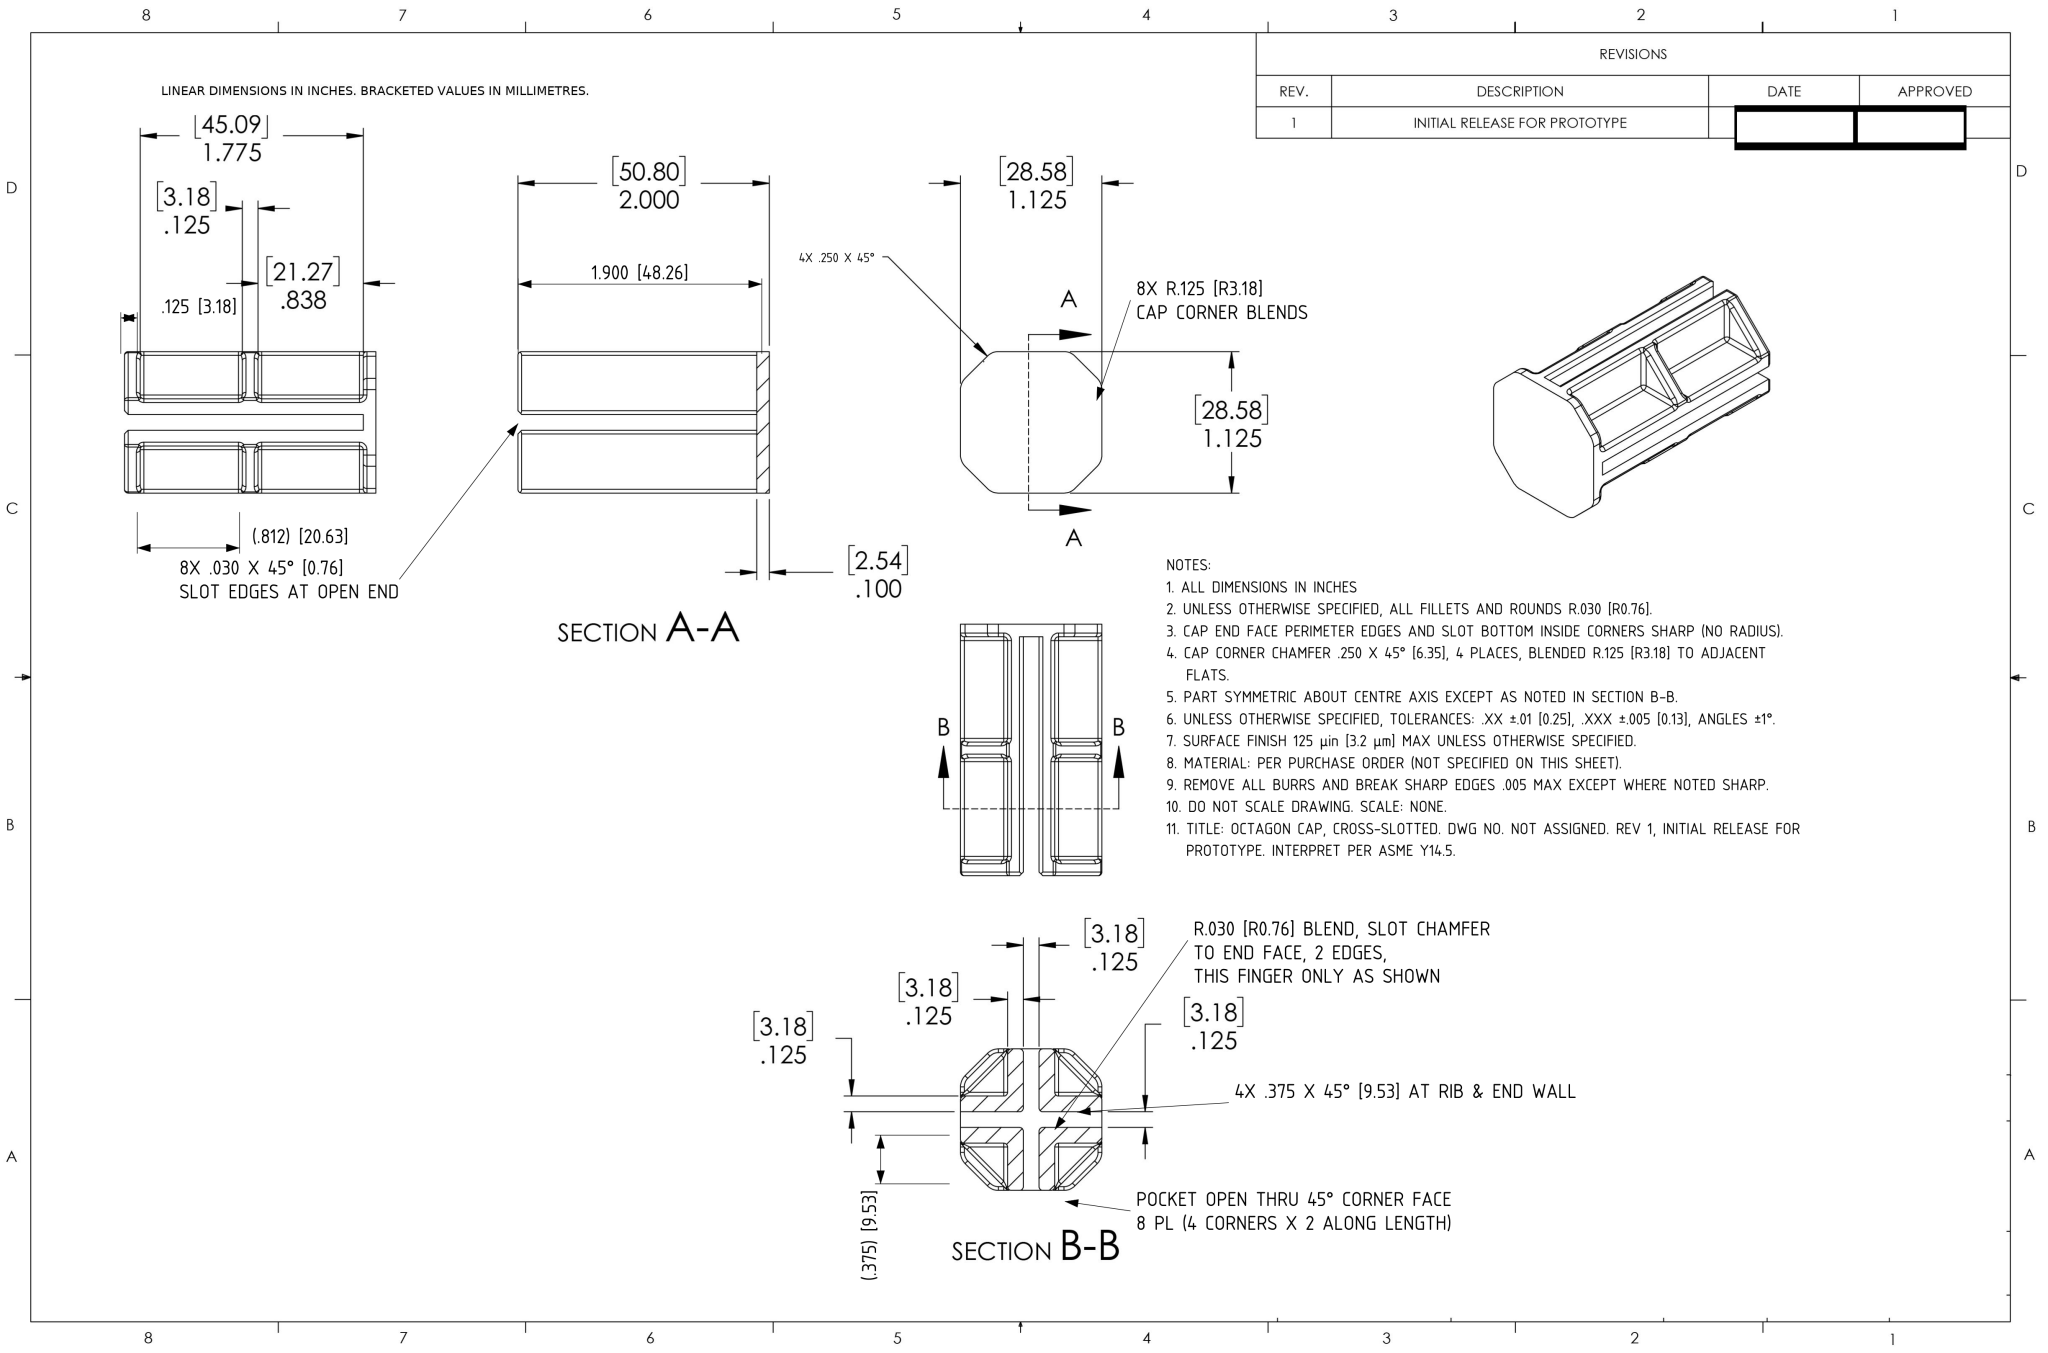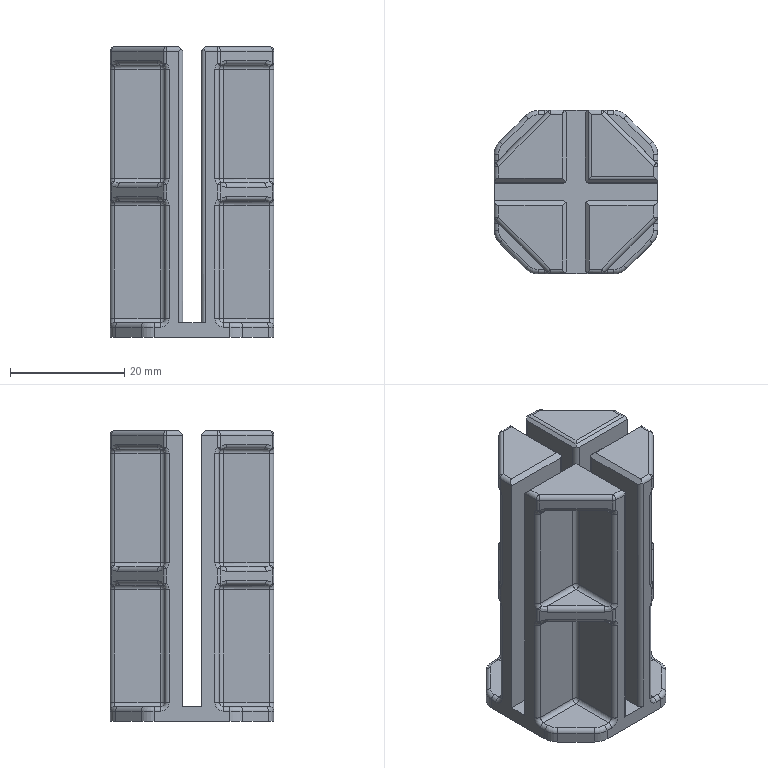Part | NX | drawing in metres | 1 solid | 308 faces | box 28.58 x 28.58 x 50.8 mm | volume 16543 mm3 | cylinder 126 | plane 70 | sphere 48 | torus 40 | spline 24 | commonest cylinder face diameters 1.524 x118 6.35 x8